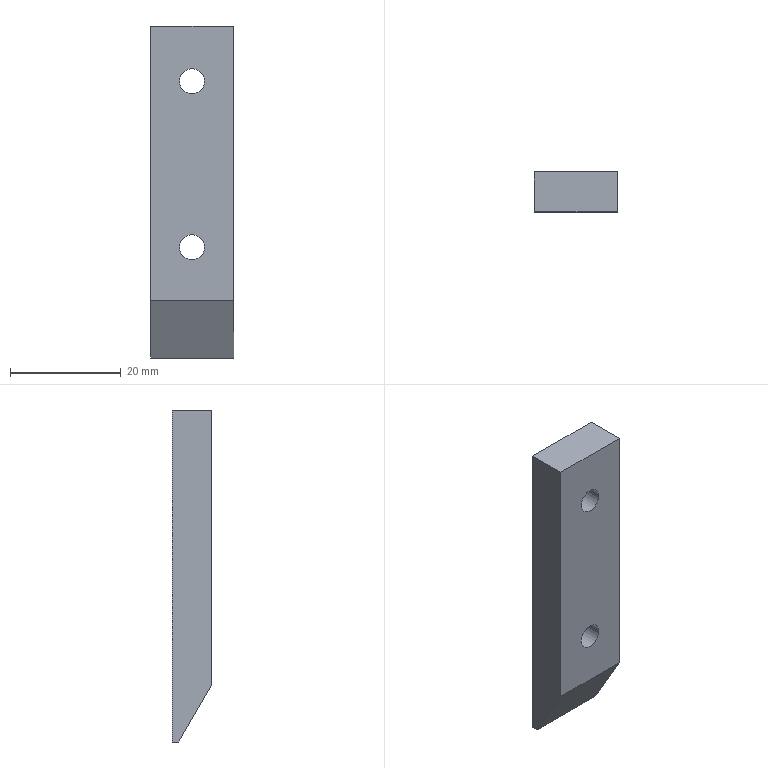Component | SolidWorks | 12-DividingMechanism-1111-1_25-1111-2 | 1 solid | 15 faces | box 15 x 7.2 x 60 mm | volume 5690 mm3 | plane 7 | cone 4 | cylinder 4 | commonest cylinder face diameters 4.5 x4
build123d program:
from build123d import *

# Parameters (mm, degrees)
SKETCH5_W                                            = 60
SKETCH5_H                                            = 15
BOSS_EXTRUDE1_DEPTH                                  = 7.2
CHAMFER1_SIZE                                        = 6
CHAMFER1_SIZE2                                       = 10.392
M4_HEXAGON_SOCKET_COUNTERSUNK_HEAD_SCREW_D           = 4.5
M4_HEXAGON_SOCKET_COUNTERSUNK_HEAD_SCREW_CSINK_D     = 8.96
M4_HEXAGON_SOCKET_COUNTERSUNK_HEAD_SCREW_CSINK_ANGLE = 90


with BuildPart() as part:
    # Sketch5 → Boss-Extrude1 (new body)
    with BuildSketch(Plane(origin=(0, 0, 0), x_dir=(1, 0, 0), z_dir=(0, 1, 0))):
        Rectangle(SKETCH5_W, SKETCH5_H)
    extrude(amount=BOSS_EXTRUDE1_DEPTH)

    # Chamfer1
    chamfer1_edges = [part.edges().sort_by_distance(p)[0] for p in [
        (30, 0, 0),
    ]]
    chamfer1_side = [part.faces().sort_by_distance(p)[0] for p in [
        (30, 3.6, 0),
    ]]
    chamfer(chamfer1_edges, length=CHAMFER1_SIZE, length2=CHAMFER1_SIZE2, reference=chamfer1_side[0])

    # M4 Hexagon Socket Countersunk Head Screw (through all)
    with Locations(Plane(origin=(0, 7.2, 0), x_dir=(1, 0, 0), z_dir=(0, 1, 0))):
        with Locations((-20, 0), (10, 0)):
            CounterSinkHole(M4_HEXAGON_SOCKET_COUNTERSUNK_HEAD_SCREW_D / 2, M4_HEXAGON_SOCKET_COUNTERSUNK_HEAD_SCREW_CSINK_D / 2, counter_sink_angle=M4_HEXAGON_SOCKET_COUNTERSUNK_HEAD_SCREW_CSINK_ANGLE)


solid = part.part

# Placed as in the assembly
solid = solid.moved(Location((-90.322, 571.824, 1524.056), (0, 90, 0)))
STEP:
#1=COLOUR_RGB('',0.7922,0.8196,0.9333);
#2=FILL_AREA_STYLE_COLOUR('',#1);
#3=FILL_AREA_STYLE('',(#2));
#4=SURFACE_STYLE_FILL_AREA(#3);
#5=SURFACE_SIDE_STYLE('',(#4));
#6=SURFACE_STYLE_USAGE(.BOTH.,#5);
#7=PRESENTATION_STYLE_ASSIGNMENT((#6));
#8=CARTESIAN_POINT('',(-3.645,22.708,60.79));
#9=VERTEX_POINT('',#8);
#10=CARTESIAN_POINT('',(-3.467,22.708,60.79));
#11=VERTEX_POINT('',#10);
#12=CARTESIAN_POINT('',(-3.556,22.708,60.79));
#13=DIRECTION('',(0.,1.,0.));
#14=DIRECTION('',(1.,0.,0.));
#15=AXIS2_PLACEMENT_3D('',#12,#13,#14);
#16=CIRCLE('',#15,0.08858);
#17=EDGE_CURVE('',#9,#11,#16,.T.);
#18=ORIENTED_EDGE('',*,*,#17,.F.);
#19=CARTESIAN_POINT('',(-3.732,22.796,60.79));
#20=VERTEX_POINT('',#19);
#21=CARTESIAN_POINT('',(-3.732,22.796,60.79));
#22=DIRECTION('',(-0.7071,0.7071,-0.));
#23=VECTOR('',#22,39.37);
#24=LINE('',#21,#23);
#25=EDGE_CURVE('',#9,#20,#24,.T.);
#26=ORIENTED_EDGE('',*,*,#25,.T.);
#27=CARTESIAN_POINT('',(-3.38,22.796,60.79));
#28=VERTEX_POINT('',#27);
#29=CARTESIAN_POINT('',(-3.556,22.796,60.79));
#30=DIRECTION('',(0.,1.,0.));
#31=DIRECTION('',(1.,0.,0.));
#32=AXIS2_PLACEMENT_3D('',#29,#30,#31);
#33=CIRCLE('',#32,0.1764);
#34=EDGE_CURVE('',#20,#28,#33,.T.);
#35=ORIENTED_EDGE('',*,*,#34,.T.);
#36=CARTESIAN_POINT('',(-3.38,22.796,60.79));
#37=DIRECTION('',(0.7071,0.7071,0.));
#38=VECTOR('',#37,39.37);
#39=LINE('',#36,#38);
#40=EDGE_CURVE('',#11,#28,#39,.T.);
#41=ORIENTED_EDGE('',*,*,#40,.F.);
#42=EDGE_LOOP('',(#18,#26,#35,#41));
#43=FACE_OUTER_BOUND('',#42,.T.);
#44=CARTESIAN_POINT('',(-3.556,22.796,60.79));
#45=DIRECTION('',(0.,1.,0.));
#46=DIRECTION('',(1.,0.,0.));
#47=AXIS2_PLACEMENT_3D('',#44,#45,#46);
#48=CONICAL_SURFACE('',#47,0.1764,0.7854);
#49=ADVANCED_FACE('',(#43),#48,.F.);
#50=CARTESIAN_POINT('',(-3.645,22.513,60.79));
#51=VERTEX_POINT('',#50);
#52=CARTESIAN_POINT('',(-3.467,22.513,60.79));
#53=VERTEX_POINT('',#52);
#54=CARTESIAN_POINT('',(-3.556,22.513,60.79));
#55=DIRECTION('',(0.,1.,0.));
#56=DIRECTION('',(1.,0.,0.));
#57=AXIS2_PLACEMENT_3D('',#54,#55,#56);
#58=CIRCLE('',#57,0.08858);
#59=EDGE_CURVE('',#51,#53,#58,.T.);
#60=ORIENTED_EDGE('',*,*,#59,.F.);
#61=CARTESIAN_POINT('',(-3.645,22.796,60.79));
#62=DIRECTION('',(0.,1.,0.));
#63=VECTOR('',#62,39.37);
#64=LINE('',#61,#63);
#65=EDGE_CURVE('',#51,#9,#64,.T.);
#66=ORIENTED_EDGE('',*,*,#65,.T.);
#67=ORIENTED_EDGE('',*,*,#17,.T.);
#68=CARTESIAN_POINT('',(-3.467,22.796,60.79));
#69=DIRECTION('',(0.,1.,0.));
#70=VECTOR('',#69,39.37);
#71=LINE('',#68,#70);
#72=EDGE_CURVE('',#53,#11,#71,.T.);
#73=ORIENTED_EDGE('',*,*,#72,.F.);
#74=EDGE_LOOP('',(#60,#66,#67,#73));
#75=FACE_OUTER_BOUND('',#74,.T.);
#76=CARTESIAN_POINT('',(-3.556,22.796,60.79));
#77=DIRECTION('',(0.,1.,0.));
#78=DIRECTION('',(1.,0.,0.));
#79=AXIS2_PLACEMENT_3D('',#76,#77,#78);
#80=CYLINDRICAL_SURFACE('',#79,0.08858);
#81=ADVANCED_FACE('',(#75),#80,.F.);
#82=CARTESIAN_POINT('',(-3.645,22.708,59.608));
#83=VERTEX_POINT('',#82);
#84=CARTESIAN_POINT('',(-3.467,22.708,59.608));
#85=VERTEX_POINT('',#84);
#86=CARTESIAN_POINT('',(-3.556,22.708,59.608));
#87=DIRECTION('',(0.,1.,0.));
#88=DIRECTION('',(1.,0.,0.));
#89=AXIS2_PLACEMENT_3D('',#86,#87,#88);
#90=CIRCLE('',#89,0.08858);
#91=EDGE_CURVE('',#83,#85,#90,.T.);
#92=ORIENTED_EDGE('',*,*,#91,.F.);
#93=CARTESIAN_POINT('',(-3.732,22.796,59.608));
#94=VERTEX_POINT('',#93);
#95=CARTESIAN_POINT('',(-3.732,22.796,59.608));
#96=DIRECTION('',(-0.7071,0.7071,-0.));
#97=VECTOR('',#96,39.37);
#98=LINE('',#95,#97);
#99=EDGE_CURVE('',#83,#94,#98,.T.);
#100=ORIENTED_EDGE('',*,*,#99,.T.);
#101=CARTESIAN_POINT('',(-3.38,22.796,59.608));
#102=VERTEX_POINT('',#101);
#103=CARTESIAN_POINT('',(-3.556,22.796,59.608));
#104=DIRECTION('',(0.,1.,0.));
#105=DIRECTION('',(1.,0.,0.));
#106=AXIS2_PLACEMENT_3D('',#103,#104,#105);
#107=CIRCLE('',#106,0.1764);
#108=EDGE_CURVE('',#94,#102,#107,.T.);
#109=ORIENTED_EDGE('',*,*,#108,.T.);
#110=CARTESIAN_POINT('',(-3.38,22.796,59.608));
#111=DIRECTION('',(0.7071,0.7071,0.));
#112=VECTOR('',#111,39.37);
#113=LINE('',#110,#112);
#114=EDGE_CURVE('',#85,#102,#113,.T.);
#115=ORIENTED_EDGE('',*,*,#114,.F.);
#116=EDGE_LOOP('',(#92,#100,#109,#115));
#117=FACE_OUTER_BOUND('',#116,.T.);
#118=CARTESIAN_POINT('',(-3.556,22.796,59.608));
#119=DIRECTION('',(0.,1.,0.));
#120=DIRECTION('',(1.,0.,0.));
#121=AXIS2_PLACEMENT_3D('',#118,#119,#120);
#122=CONICAL_SURFACE('',#121,0.1764,0.7854);
#123=ADVANCED_FACE('',(#117),#122,.F.);
#124=CARTESIAN_POINT('',(-3.645,22.513,59.608));
#125=VERTEX_POINT('',#124);
#126=CARTESIAN_POINT('',(-3.467,22.513,59.608));
#127=VERTEX_POINT('',#126);
#128=CARTESIAN_POINT('',(-3.556,22.513,59.608));
#129=DIRECTION('',(0.,1.,0.));
#130=DIRECTION('',(1.,0.,0.));
#131=AXIS2_PLACEMENT_3D('',#128,#129,#130);
#132=CIRCLE('',#131,0.08858);
#133=EDGE_CURVE('',#125,#127,#132,.T.);
#134=ORIENTED_EDGE('',*,*,#133,.F.);
#135=CARTESIAN_POINT('',(-3.645,22.796,59.608));
#136=DIRECTION('',(0.,1.,0.));
#137=VECTOR('',#136,39.37);
#138=LINE('',#135,#137);
#139=EDGE_CURVE('',#125,#83,#138,.T.);
#140=ORIENTED_EDGE('',*,*,#139,.T.);
#141=ORIENTED_EDGE('',*,*,#91,.T.);
#142=CARTESIAN_POINT('',(-3.467,22.796,59.608));
#143=DIRECTION('',(0.,1.,0.));
#144=VECTOR('',#143,39.37);
#145=LINE('',#142,#144);
#146=EDGE_CURVE('',#127,#85,#145,.T.);
#147=ORIENTED_EDGE('',*,*,#146,.F.);
#148=EDGE_LOOP('',(#134,#140,#141,#147));
#149=FACE_OUTER_BOUND('',#148,.T.);
#150=CARTESIAN_POINT('',(-3.556,22.796,59.608));
#151=DIRECTION('',(0.,1.,0.));
#152=DIRECTION('',(1.,0.,0.));
#153=AXIS2_PLACEMENT_3D('',#150,#151,#152);
#154=CYLINDRICAL_SURFACE('',#153,0.08858);
#155=ADVANCED_FACE('',(#149),#154,.F.);
#156=CARTESIAN_POINT('',(-3.851,22.513,61.183));
#157=VERTEX_POINT('',#156);
#158=CARTESIAN_POINT('',(-3.261,22.513,61.183));
#159=VERTEX_POINT('',#158);
#160=CARTESIAN_POINT('',(-3.261,22.513,61.183));
#161=DIRECTION('',(1.,-0.,0.));
#162=VECTOR('',#161,39.37);
#163=LINE('',#160,#162);
#164=EDGE_CURVE('',#157,#159,#163,.T.);
#165=ORIENTED_EDGE('',*,*,#164,.T.);
#166=CARTESIAN_POINT('',(-3.261,22.796,61.183));
#167=VERTEX_POINT('',#166);
#168=CARTESIAN_POINT('',(-3.261,22.796,61.183));
#169=DIRECTION('',(-0.,-1.,-0.));
#170=VECTOR('',#169,39.37);
#171=LINE('',#168,#170);
#172=EDGE_CURVE('',#167,#159,#171,.T.);
#173=ORIENTED_EDGE('',*,*,#172,.F.);
#174=CARTESIAN_POINT('',(-3.851,22.796,61.183));
#175=VERTEX_POINT('',#174);
#176=CARTESIAN_POINT('',(-3.261,22.796,61.183));
#177=DIRECTION('',(1.,-0.,0.));
#178=VECTOR('',#177,39.37);
#179=LINE('',#176,#178);
#180=EDGE_CURVE('',#175,#167,#179,.T.);
#181=ORIENTED_EDGE('',*,*,#180,.F.);
#182=CARTESIAN_POINT('',(-3.851,22.796,61.183));
#183=DIRECTION('',(-0.,-1.,-0.));
#184=VECTOR('',#183,39.37);
#185=LINE('',#182,#184);
#186=EDGE_CURVE('',#175,#157,#185,.T.);
#187=ORIENTED_EDGE('',*,*,#186,.T.);
#188=EDGE_LOOP('',(#165,#173,#181,#187));
#189=FACE_OUTER_BOUND('',#188,.T.);
#190=CARTESIAN_POINT('',(-3.261,22.796,61.183));
#191=DIRECTION('',(0.,0.,-1.));
#192=DIRECTION('',(-1.,0.,-0.));
#193=AXIS2_PLACEMENT_3D('',#190,#191,#192);
#194=PLANE('',#193);
#195=ADVANCED_FACE('',(#189),#194,.F.);
#196=CARTESIAN_POINT('',(-3.261,22.513,59.23));
#197=VERTEX_POINT('',#196);
#198=CARTESIAN_POINT('',(-3.261,22.513,58.821));
#199=DIRECTION('',(0.,0.,-1.));
#200=VECTOR('',#199,39.37);
#201=LINE('',#198,#200);
#202=EDGE_CURVE('',#159,#197,#201,.T.);
#203=ORIENTED_EDGE('',*,*,#202,.T.);
#204=CARTESIAN_POINT('',(-3.261,22.749,58.821));
#205=VERTEX_POINT('',#204);
#206=CARTESIAN_POINT('',(-3.261,22.749,58.821));
#207=DIRECTION('',(0.,0.5,-0.866));
#208=VECTOR('',#207,39.37);
#209=LINE('',#206,#208);
#210=EDGE_CURVE('',#197,#205,#209,.T.);
#211=ORIENTED_EDGE('',*,*,#210,.T.);
#212=CARTESIAN_POINT('',(-3.261,22.796,58.821));
#213=VERTEX_POINT('',#212);
#214=CARTESIAN_POINT('',(-3.261,22.796,58.821));
#215=DIRECTION('',(-0.,-1.,-0.));
#216=VECTOR('',#215,39.37);
#217=LINE('',#214,#216);
#218=EDGE_CURVE('',#213,#205,#217,.T.);
#219=ORIENTED_EDGE('',*,*,#218,.F.);
#220=CARTESIAN_POINT('',(-3.261,22.796,58.821));
#221=DIRECTION('',(0.,0.,-1.));
#222=VECTOR('',#221,39.37);
#223=LINE('',#220,#222);
#224=EDGE_CURVE('',#167,#213,#223,.T.);
#225=ORIENTED_EDGE('',*,*,#224,.F.);
#226=ORIENTED_EDGE('',*,*,#172,.T.);
#227=EDGE_LOOP('',(#203,#211,#219,#225,#226));
#228=FACE_OUTER_BOUND('',#227,.T.);
#229=CARTESIAN_POINT('',(-3.261,22.796,58.821));
#230=DIRECTION('',(-1.,0.,-0.));
#231=DIRECTION('',(-0.,-0.,1.));
#232=AXIS2_PLACEMENT_3D('',#229,#230,#231);
#233=PLANE('',#232);
#234=ADVANCED_FACE('',(#228),#233,.F.);
#235=ORIENTED_EDGE('',*,*,#218,.T.);
#236=CARTESIAN_POINT('',(-3.851,22.749,58.821));
#237=VERTEX_POINT('',#236);
#238=CARTESIAN_POINT('',(-3.261,22.749,58.821));
#239=DIRECTION('',(-1.,0.,-0.));
#240=VECTOR('',#239,39.37);
#241=LINE('',#238,#240);
#242=EDGE_CURVE('',#205,#237,#241,.T.);
#243=ORIENTED_EDGE('',*,*,#242,.T.);
#244=CARTESIAN_POINT('',(-3.851,22.796,58.821));
#245=VERTEX_POINT('',#244);
#246=CARTESIAN_POINT('',(-3.851,22.796,58.821));
#247=DIRECTION('',(-0.,-1.,-0.));
#248=VECTOR('',#247,39.37);
#249=LINE('',#246,#248);
#250=EDGE_CURVE('',#245,#237,#249,.T.);
#251=ORIENTED_EDGE('',*,*,#250,.F.);
#252=CARTESIAN_POINT('',(-3.261,22.796,58.821));
#253=DIRECTION('',(-1.,0.,-0.));
#254=VECTOR('',#253,39.37);
#255=LINE('',#252,#254);
#256=EDGE_CURVE('',#213,#245,#255,.T.);
#257=ORIENTED_EDGE('',*,*,#256,.F.);
#258=EDGE_LOOP('',(#235,#243,#251,#257));
#259=FACE_OUTER_BOUND('',#258,.T.);
#260=CARTESIAN_POINT('',(-3.261,22.796,58.821));
#261=DIRECTION('',(-0.,-0.,1.));
#262=DIRECTION('',(1.,-0.,0.));
#263=AXIS2_PLACEMENT_3D('',#260,#261,#262);
#264=PLANE('',#263);
#265=ADVANCED_FACE('',(#259),#264,.F.);
#266=ORIENTED_EDGE('',*,*,#250,.T.);
#267=CARTESIAN_POINT('',(-3.851,22.513,59.23));
#268=VERTEX_POINT('',#267);
#269=CARTESIAN_POINT('',(-3.851,22.749,58.821));
#270=DIRECTION('',(-0.,-0.5,0.866));
#271=VECTOR('',#270,39.37);
#272=LINE('',#269,#271);
#273=EDGE_CURVE('',#237,#268,#272,.T.);
#274=ORIENTED_EDGE('',*,*,#273,.T.);
#275=CARTESIAN_POINT('',(-3.851,22.513,58.821));
#276=DIRECTION('',(-0.,-0.,1.));
#277=VECTOR('',#276,39.37);
#278=LINE('',#275,#277);
#279=EDGE_CURVE('',#268,#157,#278,.T.);
#280=ORIENTED_EDGE('',*,*,#279,.T.);
#281=ORIENTED_EDGE('',*,*,#186,.F.);
#282=CARTESIAN_POINT('',(-3.851,22.796,58.821));
#283=DIRECTION('',(-0.,-0.,1.));
#284=VECTOR('',#283,39.37);
#285=LINE('',#282,#284);
#286=EDGE_CURVE('',#245,#175,#285,.T.);
#287=ORIENTED_EDGE('',*,*,#286,.F.);
#288=EDGE_LOOP('',(#266,#274,#280,#281,#287));
#289=FACE_OUTER_BOUND('',#288,.T.);
#290=CARTESIAN_POINT('',(-3.851,22.796,58.821));
#291=DIRECTION('',(1.,-0.,0.));
#292=DIRECTION('',(0.,0.,-1.));
#293=AXIS2_PLACEMENT_3D('',#290,#291,#292);
#294=PLANE('',#293);
#295=ADVANCED_FACE('',(#289),#294,.F.);
#296=CARTESIAN_POINT('',(-3.556,22.796,60.79));
#297=DIRECTION('',(0.,1.,0.));
#298=DIRECTION('',(1.,0.,0.));
#299=AXIS2_PLACEMENT_3D('',#296,#297,#298);
#300=CIRCLE('',#299,0.1764);
#301=EDGE_CURVE('',#28,#20,#300,.T.);
#302=ORIENTED_EDGE('',*,*,#301,.F.);
#303=ORIENTED_EDGE('',*,*,#34,.F.);
#304=EDGE_LOOP('',(#302,#303));
#305=FACE_BOUND('',#304,.T.);
#306=CARTESIAN_POINT('',(-3.556,22.796,59.608));
#307=DIRECTION('',(0.,1.,0.));
#308=DIRECTION('',(1.,0.,0.));
#309=AXIS2_PLACEMENT_3D('',#306,#307,#308);
#310=CIRCLE('',#309,0.1764);
#311=EDGE_CURVE('',#102,#94,#310,.T.);
#312=ORIENTED_EDGE('',*,*,#311,.F.);
#313=ORIENTED_EDGE('',*,*,#108,.F.);
#314=EDGE_LOOP('',(#312,#313));
#315=FACE_BOUND('',#314,.T.);
#316=ORIENTED_EDGE('',*,*,#180,.T.);
#317=ORIENTED_EDGE('',*,*,#224,.T.);
#318=ORIENTED_EDGE('',*,*,#256,.T.);
#319=ORIENTED_EDGE('',*,*,#286,.T.);
#320=EDGE_LOOP('',(#316,#317,#318,#319));
#321=FACE_OUTER_BOUND('',#320,.T.);
#322=CARTESIAN_POINT('',(-3.556,22.796,60.002));
#323=DIRECTION('',(0.,1.,0.));
#324=DIRECTION('',(1.,-0.,0.));
#325=AXIS2_PLACEMENT_3D('',#322,#323,#324);
#326=PLANE('',#325);
#327=ADVANCED_FACE('',(#305,#315,#321),#326,.T.);
#328=CARTESIAN_POINT('',(-3.556,22.513,60.79));
#329=DIRECTION('',(0.,1.,0.));
#330=DIRECTION('',(1.,0.,0.));
#331=AXIS2_PLACEMENT_3D('',#328,#329,#330);
#332=CIRCLE('',#331,0.08858);
#333=EDGE_CURVE('',#53,#51,#332,.T.);
#334=ORIENTED_EDGE('',*,*,#333,.T.);
#335=ORIENTED_EDGE('',*,*,#59,.T.);
#336=EDGE_LOOP('',(#334,#335));
#337=FACE_BOUND('',#336,.T.);
#338=CARTESIAN_POINT('',(-3.556,22.513,59.608));
#339=DIRECTION('',(0.,1.,0.));
#340=DIRECTION('',(1.,0.,0.));
#341=AXIS2_PLACEMENT_3D('',#338,#339,#340);
#342=CIRCLE('',#341,0.08858);
#343=EDGE_CURVE('',#127,#125,#342,.T.);
#344=ORIENTED_EDGE('',*,*,#343,.T.);
#345=ORIENTED_EDGE('',*,*,#133,.T.);
#346=EDGE_LOOP('',(#344,#345));
#347=FACE_BOUND('',#346,.T.);
#348=ORIENTED_EDGE('',*,*,#279,.F.);
#349=CARTESIAN_POINT('',(-3.556,22.513,59.23));
#350=DIRECTION('',(1.,-0.,0.));
#351=VECTOR('',#350,39.37);
#352=LINE('',#349,#351);
#353=EDGE_CURVE('',#268,#197,#352,.T.);
#354=ORIENTED_EDGE('',*,*,#353,.T.);
#355=ORIENTED_EDGE('',*,*,#202,.F.);
#356=ORIENTED_EDGE('',*,*,#164,.F.);
#357=EDGE_LOOP('',(#348,#354,#355,#356));
#358=FACE_OUTER_BOUND('',#357,.T.);
#359=CARTESIAN_POINT('',(-3.556,22.513,60.002));
#360=DIRECTION('',(0.,1.,0.));
#361=DIRECTION('',(1.,-0.,0.));
#362=AXIS2_PLACEMENT_3D('',#359,#360,#361);
#363=PLANE('',#362);
#364=ADVANCED_FACE('',(#337,#347,#358),#363,.F.);
#365=ORIENTED_EDGE('',*,*,#210,.F.);
#366=ORIENTED_EDGE('',*,*,#353,.F.);
#367=ORIENTED_EDGE('',*,*,#273,.F.);
#368=ORIENTED_EDGE('',*,*,#242,.F.);
#369=EDGE_LOOP('',(#365,#366,#367,#368));
#370=FACE_OUTER_BOUND('',#369,.T.);
#371=CARTESIAN_POINT('',(-3.261,22.749,58.821));
#372=DIRECTION('',(-0.,0.866,0.5));
#373=DIRECTION('',(-1.,0.,-0.));
#374=AXIS2_PLACEMENT_3D('',#371,#372,#373);
#375=PLANE('',#374);
#376=ADVANCED_FACE('',(#370),#375,.F.);
#377=ORIENTED_EDGE('',*,*,#139,.F.);
#378=ORIENTED_EDGE('',*,*,#343,.F.);
#379=ORIENTED_EDGE('',*,*,#146,.T.);
#380=CARTESIAN_POINT('',(-3.556,22.708,59.608));
#381=DIRECTION('',(0.,1.,0.));
#382=DIRECTION('',(1.,0.,0.));
#383=AXIS2_PLACEMENT_3D('',#380,#381,#382);
#384=CIRCLE('',#383,0.08858);
#385=EDGE_CURVE('',#85,#83,#384,.T.);
#386=ORIENTED_EDGE('',*,*,#385,.T.);
#387=EDGE_LOOP('',(#377,#378,#379,#386));
#388=FACE_OUTER_BOUND('',#387,.T.);
#389=CARTESIAN_POINT('',(-3.556,22.796,59.608));
#390=DIRECTION('',(0.,1.,0.));
#391=DIRECTION('',(1.,0.,0.));
#392=AXIS2_PLACEMENT_3D('',#389,#390,#391);
#393=CYLINDRICAL_SURFACE('',#392,0.08858);
#394=ADVANCED_FACE('',(#388),#393,.F.);
#395=ORIENTED_EDGE('',*,*,#99,.F.);
#396=ORIENTED_EDGE('',*,*,#385,.F.);
#397=ORIENTED_EDGE('',*,*,#114,.T.);
#398=ORIENTED_EDGE('',*,*,#311,.T.);
#399=EDGE_LOOP('',(#395,#396,#397,#398));
#400=FACE_OUTER_BOUND('',#399,.T.);
#401=CARTESIAN_POINT('',(-3.556,22.796,59.608));
#402=DIRECTION('',(0.,1.,0.));
#403=DIRECTION('',(1.,0.,0.));
#404=AXIS2_PLACEMENT_3D('',#401,#402,#403);
#405=CONICAL_SURFACE('',#404,0.1764,0.7854);
#406=ADVANCED_FACE('',(#400),#405,.F.);
#407=ORIENTED_EDGE('',*,*,#65,.F.);
#408=ORIENTED_EDGE('',*,*,#333,.F.);
#409=ORIENTED_EDGE('',*,*,#72,.T.);
#410=CARTESIAN_POINT('',(-3.556,22.708,60.79));
#411=DIRECTION('',(0.,1.,0.));
#412=DIRECTION('',(1.,0.,0.));
#413=AXIS2_PLACEMENT_3D('',#410,#411,#412);
#414=CIRCLE('',#413,0.08858);
#415=EDGE_CURVE('',#11,#9,#414,.T.);
#416=ORIENTED_EDGE('',*,*,#415,.T.);
#417=EDGE_LOOP('',(#407,#408,#409,#416));
#418=FACE_OUTER_BOUND('',#417,.T.);
#419=CARTESIAN_POINT('',(-3.556,22.796,60.79));
#420=DIRECTION('',(0.,1.,0.));
#421=DIRECTION('',(1.,0.,0.));
#422=AXIS2_PLACEMENT_3D('',#419,#420,#421);
#423=CYLINDRICAL_SURFACE('',#422,0.08858);
#424=ADVANCED_FACE('',(#418),#423,.F.);
#425=ORIENTED_EDGE('',*,*,#25,.F.);
#426=ORIENTED_EDGE('',*,*,#415,.F.);
#427=ORIENTED_EDGE('',*,*,#40,.T.);
#428=ORIENTED_EDGE('',*,*,#301,.T.);
#429=EDGE_LOOP('',(#425,#426,#427,#428));
#430=FACE_OUTER_BOUND('',#429,.T.);
#431=CARTESIAN_POINT('',(-3.556,22.796,60.79));
#432=DIRECTION('',(0.,1.,0.));
#433=DIRECTION('',(1.,0.,0.));
#434=AXIS2_PLACEMENT_3D('',#431,#432,#433);
#435=CONICAL_SURFACE('',#434,0.1764,0.7854);
#436=ADVANCED_FACE('',(#430),#435,.F.);
#437=CLOSED_SHELL('',(#49,#81,#123,#155,#195,#234,#265,#295,#327,#364,#376,#394,#406,#424,#436));
#438=MANIFOLD_SOLID_BREP('',#437);
#439=STYLED_ITEM('',(#7),#438);
#440=PRESENTATION_LAYER_ASSIGNMENT('','',(#439));
#441=(LENGTH_UNIT()NAMED_UNIT(*)SI_UNIT($,.METRE.));
#442=LENGTH_MEASURE_WITH_UNIT(LENGTH_MEASURE(0.0254),#441);
#443=DIMENSIONAL_EXPONENTS(1.,0.,0.,0.,0.,0.,0.);
#444=(CONVERSION_BASED_UNIT('',#442)LENGTH_UNIT()NAMED_UNIT(#443));
#445=UNCERTAINTY_MEASURE_WITH_UNIT(LENGTH_MEASURE(0.00001),#444,'','');
#446=(NAMED_UNIT(*)PLANE_ANGLE_UNIT()SI_UNIT($,.RADIAN.));
#447=(NAMED_UNIT(*)SI_UNIT($,.STERADIAN.)SOLID_ANGLE_UNIT());
#448=(GEOMETRIC_REPRESENTATION_CONTEXT(3)GLOBAL_UNCERTAINTY_ASSIGNED_CONTEXT((#445))GLOBAL_UNIT_ASSIGNED_CONTEXT((#444,#446,#447))REPRESENTATION_CONTEXT('',''));
#449=MECHANICAL_DESIGN_GEOMETRIC_PRESENTATION_REPRESENTATION('',(#439),#448);
#450=CARTESIAN_POINT('',(0.,0.,0.));
#451=DIRECTION('',(0.,0.,1.));
#452=DIRECTION('',(1.,0.,0.));
#453=AXIS2_PLACEMENT_3D('',#450,#451,#452);
#454=(LENGTH_UNIT()NAMED_UNIT(*)SI_UNIT($,.METRE.));
#455=LENGTH_MEASURE_WITH_UNIT(LENGTH_MEASURE(0.0254),#454);
#456=DIMENSIONAL_EXPONENTS(1.,0.,0.,0.,0.,0.,0.);
#457=(CONVERSION_BASED_UNIT('',#455)LENGTH_UNIT()NAMED_UNIT(#456));
#458=UNCERTAINTY_MEASURE_WITH_UNIT(LENGTH_MEASURE(0.00001),#457,'','');
#459=(NAMED_UNIT(*)PLANE_ANGLE_UNIT()SI_UNIT($,.RADIAN.));
#460=(NAMED_UNIT(*)SI_UNIT($,.STERADIAN.)SOLID_ANGLE_UNIT());
#461=(GEOMETRIC_REPRESENTATION_CONTEXT(3)GLOBAL_UNCERTAINTY_ASSIGNED_CONTEXT((#458))GLOBAL_UNIT_ASSIGNED_CONTEXT((#457,#459,#460))REPRESENTATION_CONTEXT('',''));
#462=ADVANCED_BREP_SHAPE_REPRESENTATION('',(#438,#453),#461);